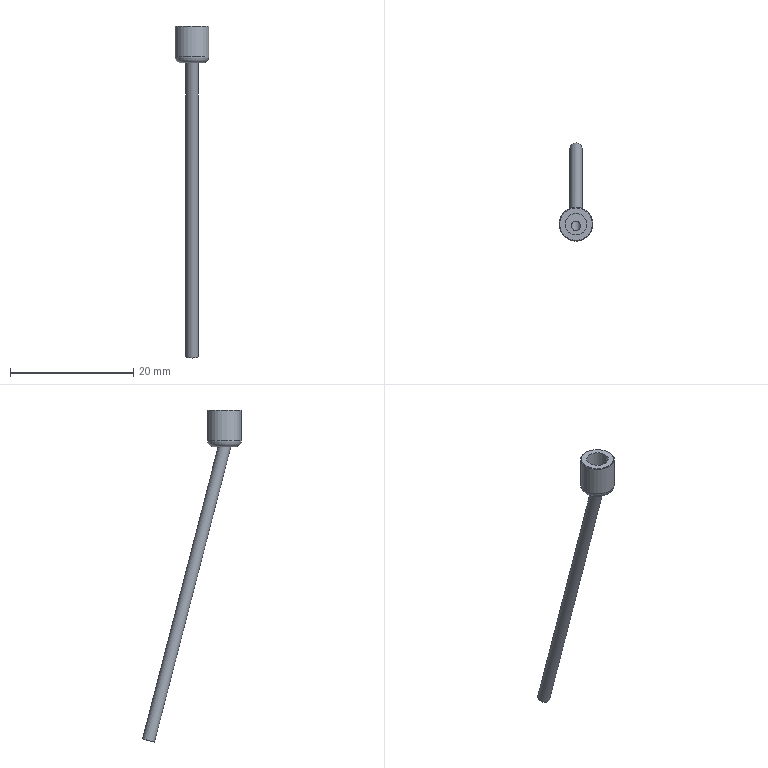Component | NX | AIR_PUMP_PART_01_12 | 1 solid | 10 faces | box 5.5 x 16.05 x 53.95 mm | volume 157 mm3 | plane 4 | cylinder 4 | torus 1 | cone 1 | commonest cylinder face diameters 5.5 x1 2 x1 1.5 x1 3.5 x1
STEP:
#1=CARTESIAN_POINT('',(0.,0.,0.));
#2=DIRECTION('',(0.,0.,1.));
#3=DIRECTION('',(1.,0.,0.));
#4=AXIS2_PLACEMENT_3D('',#1,#2,#3);
#5=CARTESIAN_POINT('',(0.0005589,-29.55,80.052));
#6=VERTEX_POINT('',#5);
#7=CARTESIAN_POINT('',(0.0005589,-32.2,80.052));
#8=DIRECTION('',(0.,0.,1.));
#9=DIRECTION('',(0.,1.,0.));
#10=AXIS2_PLACEMENT_3D('',#7,#8,#9);
#11=CIRCLE('',#10,2.65);
#12=CARTESIAN_POINT('',(0.0005589,-32.2,80.052));
#13=DIRECTION('',(0.,0.,1.));
#14=DIRECTION('',(0.,1.,0.));
#15=AXIS2_PLACEMENT_3D('',#12,#13,#14);
#16=PLANE('',#15);
#17=CARTESIAN_POINT('',(0.,0.));
#18=DIRECTION('',(1.,0.));
#19=AXIS2_PLACEMENT_2D('',#17,#18);
#20=CIRCLE('',#19,2.65);
#21=(GEOMETRIC_REPRESENTATION_CONTEXT(2)PARAMETRIC_REPRESENTATION_CONTEXT()REPRESENTATION_CONTEXT('',''));
#22=DEFINITIONAL_REPRESENTATION('',(#20),#21);
#23=PCURVE('',#16,#22);
#24=CARTESIAN_POINT('',(0.0005589,-32.2,79.952));
#25=DIRECTION('',(0.,0.,-1.));
#26=DIRECTION('',(0.,-1.,0.));
#27=AXIS2_PLACEMENT_3D('',#24,#25,#26);
#28=CONICAL_SURFACE('',#27,2.75,0.7854);
#29=CARTESIAN_POINT('',(9.425,-0.1));
#30=DIRECTION('',(-1.,0.));
#31=VECTOR('',#30,1.);
#32=LINE('',#29,#31);
#33=(GEOMETRIC_REPRESENTATION_CONTEXT(2)PARAMETRIC_REPRESENTATION_CONTEXT()REPRESENTATION_CONTEXT('',''));
#34=DEFINITIONAL_REPRESENTATION('',(#32),#33);
#35=PCURVE('',#28,#34);
#36=SURFACE_CURVE('',#11,(#23,#35),.PCURVE_S1.);
#37=EDGE_CURVE('',#6,#6,#36,.T.);
#38=ORIENTED_EDGE('',*,*,#37,.T.);
#39=EDGE_LOOP('',(#38));
#40=FACE_BOUND('',#39,.T.);
#41=CARTESIAN_POINT('',(0.0005589,-30.45,80.052));
#42=VERTEX_POINT('',#41);
#43=CARTESIAN_POINT('',(0.0005589,-32.2,80.052));
#44=DIRECTION('',(0.,0.,-1.));
#45=DIRECTION('',(-0.,1.,0.));
#46=AXIS2_PLACEMENT_3D('',#43,#44,#45);
#47=CIRCLE('',#46,1.75);
#48=CARTESIAN_POINT('',(1.75,0.));
#49=CARTESIAN_POINT('',(1.75,-3.031));
#50=CARTESIAN_POINT('',(-0.875,-1.516));
#51=CARTESIAN_POINT('',(-3.5,-0.));
#52=CARTESIAN_POINT('',(-0.875,1.516));
#53=CARTESIAN_POINT('',(1.75,3.031));
#54=CARTESIAN_POINT('',(1.75,0.));
#55=(BOUNDED_CURVE()B_SPLINE_CURVE(2,(#48,#49,#50,#51,#52,#53,#54),.UNSPECIFIED.,.T.,.F.)B_SPLINE_CURVE_WITH_KNOTS((1,2,2,2,2,1),(-2.094,0.,2.094,4.189,6.283,8.378),.UNSPECIFIED.)CURVE()GEOMETRIC_REPRESENTATION_ITEM()RATIONAL_B_SPLINE_CURVE((1.,0.5,1.,0.5,1.,0.5,1.))REPRESENTATION_ITEM(''));
#56=(GEOMETRIC_REPRESENTATION_CONTEXT(2)PARAMETRIC_REPRESENTATION_CONTEXT()REPRESENTATION_CONTEXT('',''));
#57=DEFINITIONAL_REPRESENTATION('',(#55),#56);
#58=PCURVE('',#16,#57);
#59=CARTESIAN_POINT('',(0.0005589,-32.2,75.052));
#60=DIRECTION('',(0.,0.,1.));
#61=DIRECTION('',(0.,1.,0.));
#62=AXIS2_PLACEMENT_3D('',#59,#60,#61);
#63=CYLINDRICAL_SURFACE('',#62,1.75);
#64=CARTESIAN_POINT('',(6.283,5.));
#65=DIRECTION('',(-1.,0.));
#66=VECTOR('',#65,1.);
#67=LINE('',#64,#66);
#68=(GEOMETRIC_REPRESENTATION_CONTEXT(2)PARAMETRIC_REPRESENTATION_CONTEXT()REPRESENTATION_CONTEXT('',''));
#69=DEFINITIONAL_REPRESENTATION('',(#67),#68);
#70=PCURVE('',#63,#69);
#71=SURFACE_CURVE('',#47,(#58,#70),.PCURVE_S1.);
#72=EDGE_CURVE('',#42,#42,#71,.T.);
#73=ORIENTED_EDGE('',*,*,#72,.T.);
#74=EDGE_LOOP('',(#73));
#75=FACE_BOUND('',#74,.T.);
#76=ADVANCED_FACE('',(#40,#75),#16,.T.);
#77=CARTESIAN_POINT('',(0.0005589,-33.95,74.052));
#78=VERTEX_POINT('',#77);
#79=CARTESIAN_POINT('',(0.0005589,-32.2,74.052));
#80=DIRECTION('',(0.,0.,-1.));
#81=DIRECTION('',(0.,-1.,0.));
#82=AXIS2_PLACEMENT_3D('',#79,#80,#81);
#83=CIRCLE('',#82,1.75);
#84=CARTESIAN_POINT('',(0.0005589,-32.2,74.052));
#85=DIRECTION('',(0.,0.,-1.));
#86=DIRECTION('',(0.,-1.,0.));
#87=AXIS2_PLACEMENT_3D('',#84,#85,#86);
#88=PLANE('',#87);
#89=CARTESIAN_POINT('',(0.,0.));
#90=DIRECTION('',(1.,0.));
#91=AXIS2_PLACEMENT_2D('',#89,#90);
#92=CIRCLE('',#91,1.75);
#93=(GEOMETRIC_REPRESENTATION_CONTEXT(2)PARAMETRIC_REPRESENTATION_CONTEXT()REPRESENTATION_CONTEXT('',''));
#94=DEFINITIONAL_REPRESENTATION('',(#92),#93);
#95=PCURVE('',#88,#94);
#96=CARTESIAN_POINT('',(0.0005589,-32.2,75.052));
#97=DIRECTION('',(0.,0.,-1.));
#98=DIRECTION('',(0.,-1.,0.));
#99=AXIS2_PLACEMENT_3D('',#96,#97,#98);
#100=TOROIDAL_SURFACE('',#99,1.75,1.);
#101=CARTESIAN_POINT('',(0.,7.854));
#102=DIRECTION('',(1.,0.));
#103=VECTOR('',#102,1.);
#104=LINE('',#101,#103);
#105=(GEOMETRIC_REPRESENTATION_CONTEXT(2)PARAMETRIC_REPRESENTATION_CONTEXT()REPRESENTATION_CONTEXT('',''));
#106=DEFINITIONAL_REPRESENTATION('',(#104),#105);
#107=PCURVE('',#100,#106);
#108=SURFACE_CURVE('',#83,(#95,#107),.PCURVE_S1.);
#109=EDGE_CURVE('',#78,#78,#108,.T.);
#110=ORIENTED_EDGE('',*,*,#109,.T.);
#111=EDGE_LOOP('',(#110));
#112=FACE_BOUND('',#111,.T.);
#113=CARTESIAN_POINT('',(0.0005589,-31.167,74.052));
#114=VERTEX_POINT('',#113);
#115=CARTESIAN_POINT('',(0.0005589,-33.233,74.052));
#116=VERTEX_POINT('',#115);
#117=CARTESIAN_POINT('',(0.0005589,-32.2,74.052));
#118=DIRECTION('',(0.,0.,-1.));
#119=DIRECTION('',(0.,1.,0.));
#120=AXIS2_PLACEMENT_3D('',#117,#118,#119);
#121=ELLIPSE('',#120,1.033,1.);
#122=CARTESIAN_POINT('',(0.,0.));
#123=DIRECTION('',(-1.,0.));
#124=AXIS2_PLACEMENT_2D('',#122,#123);
#125=ELLIPSE('',#124,1.033,1.);
#126=(GEOMETRIC_REPRESENTATION_CONTEXT(2)PARAMETRIC_REPRESENTATION_CONTEXT()REPRESENTATION_CONTEXT('',''));
#127=DEFINITIONAL_REPRESENTATION('',(#125),#126);
#128=PCURVE('',#88,#127);
#129=CARTESIAN_POINT('',(0.0005589,-32.2,74.052));
#130=DIRECTION('',(0.,0.2504,-0.9681));
#131=DIRECTION('',(0.,-0.9681,-0.2504));
#132=AXIS2_PLACEMENT_3D('',#129,#130,#131);
#133=CYLINDRICAL_SURFACE('',#132,1.);
#134=CARTESIAN_POINT('',(3.142,0.2586));
#135=CARTESIAN_POINT('',(3.237,0.2588));
#136=CARTESIAN_POINT('',(3.427,0.2515));
#137=CARTESIAN_POINT('',(3.713,0.2206));
#138=CARTESIAN_POINT('',(3.998,0.1717));
#139=CARTESIAN_POINT('',(4.284,0.1089));
#140=CARTESIAN_POINT('',(4.57,0.03731));
#141=CARTESIAN_POINT('',(4.855,-0.03731));
#142=CARTESIAN_POINT('',(5.141,-0.1089));
#143=CARTESIAN_POINT('',(5.426,-0.1717));
#144=CARTESIAN_POINT('',(5.712,-0.2205));
#145=CARTESIAN_POINT('',(5.998,-0.2515));
#146=CARTESIAN_POINT('',(6.283,-0.2622));
#147=CARTESIAN_POINT('',(6.569,-0.2515));
#148=CARTESIAN_POINT('',(6.854,-0.2205));
#149=CARTESIAN_POINT('',(7.14,-0.1717));
#150=CARTESIAN_POINT('',(7.426,-0.1089));
#151=CARTESIAN_POINT('',(7.711,-0.03731));
#152=CARTESIAN_POINT('',(7.997,0.03731));
#153=CARTESIAN_POINT('',(8.282,0.1089));
#154=CARTESIAN_POINT('',(8.568,0.1717));
#155=CARTESIAN_POINT('',(8.854,0.2206));
#156=CARTESIAN_POINT('',(9.139,0.2515));
#157=CARTESIAN_POINT('',(9.33,0.2588));
#158=CARTESIAN_POINT('',(9.425,0.2586));
#159=B_SPLINE_CURVE_WITH_KNOTS('',3,(#134,#135,#136,#137,#138,#139,#140,#141,#142,#143,#144,#145,#146,#147,#148,#149,#150,#151,#152,#153,#154,#155,#156,#157,#158),.UNSPECIFIED.,.F.,.F.,(4,1,1,1,1,1,1,1,1,1,1,1,1,1,1,1,1,1,1,1,1,1,4),(0.,0.2856,0.5712,0.8568,1.142,1.428,1.714,1.999,2.285,2.57,2.856,3.142,3.427,3.713,3.998,4.284,4.57,4.855,5.141,5.426,5.712,5.998,6.283),.QUASI_UNIFORM_KNOTS.);
#160=(GEOMETRIC_REPRESENTATION_CONTEXT(2)PARAMETRIC_REPRESENTATION_CONTEXT()REPRESENTATION_CONTEXT('',''));
#161=DEFINITIONAL_REPRESENTATION('',(#159),#160);
#162=PCURVE('',#133,#161);
#163=SURFACE_CURVE('',#121,(#128,#162),.PCURVE_S1.);
#164=EDGE_CURVE('',#114,#116,#163,.T.);
#165=ORIENTED_EDGE('',*,*,#164,.F.);
#166=CARTESIAN_POINT('',(0.0005589,-32.2,74.052));
#167=DIRECTION('',(0.,0.,-1.));
#168=DIRECTION('',(0.,1.,0.));
#169=AXIS2_PLACEMENT_3D('',#166,#167,#168);
#170=ELLIPSE('',#169,1.033,1.);
#171=CARTESIAN_POINT('',(0.,0.));
#172=DIRECTION('',(-1.,0.));
#173=AXIS2_PLACEMENT_2D('',#171,#172);
#174=ELLIPSE('',#173,1.033,1.);
#175=(GEOMETRIC_REPRESENTATION_CONTEXT(2)PARAMETRIC_REPRESENTATION_CONTEXT()REPRESENTATION_CONTEXT('',''));
#176=DEFINITIONAL_REPRESENTATION('',(#174),#175);
#177=PCURVE('',#88,#176);
#178=CARTESIAN_POINT('',(-3.142,0.2586));
#179=CARTESIAN_POINT('',(-3.046,0.2588));
#180=CARTESIAN_POINT('',(-2.856,0.2515));
#181=CARTESIAN_POINT('',(-2.57,0.2206));
#182=CARTESIAN_POINT('',(-2.285,0.1717));
#183=CARTESIAN_POINT('',(-1.999,0.1089));
#184=CARTESIAN_POINT('',(-1.714,0.03731));
#185=CARTESIAN_POINT('',(-1.428,-0.03731));
#186=CARTESIAN_POINT('',(-1.142,-0.1089));
#187=CARTESIAN_POINT('',(-0.8568,-0.1717));
#188=CARTESIAN_POINT('',(-0.5712,-0.2205));
#189=CARTESIAN_POINT('',(-0.2856,-0.2515));
#190=CARTESIAN_POINT('',(0.,-0.2622));
#191=CARTESIAN_POINT('',(0.2856,-0.2515));
#192=CARTESIAN_POINT('',(0.5712,-0.2205));
#193=CARTESIAN_POINT('',(0.8568,-0.1717));
#194=CARTESIAN_POINT('',(1.142,-0.1089));
#195=CARTESIAN_POINT('',(1.428,-0.03731));
#196=CARTESIAN_POINT('',(1.714,0.03731));
#197=CARTESIAN_POINT('',(1.999,0.1089));
#198=CARTESIAN_POINT('',(2.285,0.1717));
#199=CARTESIAN_POINT('',(2.57,0.2206));
#200=CARTESIAN_POINT('',(2.856,0.2515));
#201=CARTESIAN_POINT('',(3.046,0.2588));
#202=CARTESIAN_POINT('',(3.142,0.2586));
#203=B_SPLINE_CURVE_WITH_KNOTS('',3,(#178,#179,#180,#181,#182,#183,#184,#185,#186,#187,#188,#189,#190,#191,#192,#193,#194,#195,#196,#197,#198,#199,#200,#201,#202),.UNSPECIFIED.,.F.,.F.,(4,1,1,1,1,1,1,1,1,1,1,1,1,1,1,1,1,1,1,1,1,1,4),(0.,0.2856,0.5712,0.8568,1.142,1.428,1.714,1.999,2.285,2.57,2.856,3.142,3.427,3.713,3.998,4.284,4.57,4.855,5.141,5.426,5.712,5.998,6.283),.QUASI_UNIFORM_KNOTS.);
#204=(GEOMETRIC_REPRESENTATION_CONTEXT(2)PARAMETRIC_REPRESENTATION_CONTEXT()REPRESENTATION_CONTEXT('',''));
#205=DEFINITIONAL_REPRESENTATION('',(#203),#204);
#206=PCURVE('',#133,#205);
#207=SURFACE_CURVE('',#170,(#177,#206),.PCURVE_S1.);
#208=EDGE_CURVE('',#116,#114,#207,.T.);
#209=ORIENTED_EDGE('',*,*,#208,.F.);
#210=EDGE_LOOP('',(#165,#209));
#211=FACE_BOUND('',#210,.T.);
#212=ADVANCED_FACE('',(#112,#211),#88,.T.);
#213=CARTESIAN_POINT('',(0.0005589,-29.45,79.952));
#214=VERTEX_POINT('',#213);
#215=CARTESIAN_POINT('',(0.0005589,-32.2,79.952));
#216=DIRECTION('',(0.,0.,-1.));
#217=DIRECTION('',(0.,1.,0.));
#218=AXIS2_PLACEMENT_3D('',#215,#216,#217);
#219=CIRCLE('',#218,2.75);
#220=CARTESIAN_POINT('',(0.0005589,-32.2,74.052));
#221=DIRECTION('',(0.,0.,1.));
#222=DIRECTION('',(0.,1.,0.));
#223=AXIS2_PLACEMENT_3D('',#220,#221,#222);
#224=CYLINDRICAL_SURFACE('',#223,2.75);
#225=CARTESIAN_POINT('',(6.283,5.9));
#226=DIRECTION('',(-1.,0.));
#227=VECTOR('',#226,1.);
#228=LINE('',#225,#227);
#229=(GEOMETRIC_REPRESENTATION_CONTEXT(2)PARAMETRIC_REPRESENTATION_CONTEXT()REPRESENTATION_CONTEXT('',''));
#230=DEFINITIONAL_REPRESENTATION('',(#228),#229);
#231=PCURVE('',#224,#230);
#232=CARTESIAN_POINT('',(3.142,0.));
#233=DIRECTION('',(1.,0.));
#234=VECTOR('',#233,1.);
#235=LINE('',#232,#234);
#236=(GEOMETRIC_REPRESENTATION_CONTEXT(2)PARAMETRIC_REPRESENTATION_CONTEXT()REPRESENTATION_CONTEXT('',''));
#237=DEFINITIONAL_REPRESENTATION('',(#235),#236);
#238=PCURVE('',#28,#237);
#239=SURFACE_CURVE('',#219,(#231,#238),.PCURVE_S1.);
#240=EDGE_CURVE('',#214,#214,#239,.T.);
#241=ORIENTED_EDGE('',*,*,#240,.T.);
#242=CARTESIAN_POINT('',(0.0005589,-29.45,75.052));
#243=VERTEX_POINT('',#242);
#244=CARTESIAN_POINT('',(0.0005589,-29.45,75.052));
#245=CARTESIAN_POINT('',(0.0005589,-29.45,79.952));
#246=B_SPLINE_CURVE_WITH_KNOTS('',1,(#244,#245),.UNSPECIFIED.,.F.,.F.,(2,2),(1.,5.9),.PIECEWISE_BEZIER_KNOTS.);
#247=CARTESIAN_POINT('',(0.,0.));
#248=DIRECTION('',(0.,1.));
#249=VECTOR('',#248,1.);
#250=LINE('',#247,#249);
#251=(GEOMETRIC_REPRESENTATION_CONTEXT(2)PARAMETRIC_REPRESENTATION_CONTEXT()REPRESENTATION_CONTEXT('',''));
#252=DEFINITIONAL_REPRESENTATION('',(#250),#251);
#253=PCURVE('',#224,#252);
#254=CARTESIAN_POINT('',(6.283,0.));
#255=DIRECTION('',(0.,1.));
#256=VECTOR('',#255,1.);
#257=LINE('',#254,#256);
#258=(GEOMETRIC_REPRESENTATION_CONTEXT(2)PARAMETRIC_REPRESENTATION_CONTEXT()REPRESENTATION_CONTEXT('',''));
#259=DEFINITIONAL_REPRESENTATION('',(#257),#258);
#260=PCURVE('',#224,#259);
#261=SEAM_CURVE('',#246,(#253,#260),.PCURVE_S1.);
#262=EDGE_CURVE('',#243,#214,#261,.T.);
#263=ORIENTED_EDGE('',*,*,#262,.F.);
#264=CARTESIAN_POINT('',(0.0005589,-34.95,75.052));
#265=VERTEX_POINT('',#264);
#266=CARTESIAN_POINT('',(0.0005589,-32.2,75.052));
#267=DIRECTION('',(0.,0.,1.));
#268=DIRECTION('',(0.,-1.,0.));
#269=AXIS2_PLACEMENT_3D('',#266,#267,#268);
#270=CIRCLE('',#269,2.75);
#271=CARTESIAN_POINT('',(-3.142,1.));
#272=DIRECTION('',(1.,0.));
#273=VECTOR('',#272,1.);
#274=LINE('',#271,#273);
#275=(GEOMETRIC_REPRESENTATION_CONTEXT(2)PARAMETRIC_REPRESENTATION_CONTEXT()REPRESENTATION_CONTEXT('',''));
#276=DEFINITIONAL_REPRESENTATION('',(#274),#275);
#277=PCURVE('',#224,#276);
#278=CARTESIAN_POINT('',(6.283,6.283));
#279=DIRECTION('',(-1.,0.));
#280=VECTOR('',#279,1.);
#281=LINE('',#278,#280);
#282=(GEOMETRIC_REPRESENTATION_CONTEXT(2)PARAMETRIC_REPRESENTATION_CONTEXT()REPRESENTATION_CONTEXT('',''));
#283=DEFINITIONAL_REPRESENTATION('',(#281),#282);
#284=PCURVE('',#100,#283);
#285=SURFACE_CURVE('',#270,(#277,#284),.PCURVE_S1.);
#286=EDGE_CURVE('',#243,#265,#285,.T.);
#287=ORIENTED_EDGE('',*,*,#286,.T.);
#288=CARTESIAN_POINT('',(0.0005589,-32.2,75.052));
#289=DIRECTION('',(0.,0.,1.));
#290=DIRECTION('',(0.,-1.,0.));
#291=AXIS2_PLACEMENT_3D('',#288,#289,#290);
#292=CIRCLE('',#291,2.75);
#293=CARTESIAN_POINT('',(3.142,1.));
#294=DIRECTION('',(1.,0.));
#295=VECTOR('',#294,1.);
#296=LINE('',#293,#295);
#297=(GEOMETRIC_REPRESENTATION_CONTEXT(2)PARAMETRIC_REPRESENTATION_CONTEXT()REPRESENTATION_CONTEXT('',''));
#298=DEFINITIONAL_REPRESENTATION('',(#296),#297);
#299=PCURVE('',#224,#298);
#300=CARTESIAN_POINT('',(6.283,6.283));
#301=DIRECTION('',(-1.,0.));
#302=VECTOR('',#301,1.);
#303=LINE('',#300,#302);
#304=(GEOMETRIC_REPRESENTATION_CONTEXT(2)PARAMETRIC_REPRESENTATION_CONTEXT()REPRESENTATION_CONTEXT('',''));
#305=DEFINITIONAL_REPRESENTATION('',(#303),#304);
#306=PCURVE('',#100,#305);
#307=SURFACE_CURVE('',#292,(#299,#306),.PCURVE_S1.);
#308=EDGE_CURVE('',#265,#243,#307,.T.);
#309=ORIENTED_EDGE('',*,*,#308,.T.);
#310=ORIENTED_EDGE('',*,*,#262,.T.);
#311=EDGE_LOOP('',(#241,#263,#287,#309,#310));
#312=FACE_BOUND('',#311,.T.);
#313=ADVANCED_FACE('',(#312),#224,.T.);
#314=ORIENTED_EDGE('',*,*,#164,.T.);
#315=CARTESIAN_POINT('',(0.0005589,-20.832,26.101));
#316=VERTEX_POINT('',#315);
#317=CARTESIAN_POINT('',(0.0005589,-33.233,74.052));
#318=CARTESIAN_POINT('',(0.0005589,-20.832,26.101));
#319=B_SPLINE_CURVE_WITH_KNOTS('',1,(#317,#318),.UNSPECIFIED.,.F.,.F.,(2,2),(-0.2586,49.269),.PIECEWISE_BEZIER_KNOTS.);
#320=CARTESIAN_POINT('',(6.283,0.));
#321=DIRECTION('',(0.,1.));
#322=VECTOR('',#321,1.);
#323=LINE('',#320,#322);
#324=(GEOMETRIC_REPRESENTATION_CONTEXT(2)PARAMETRIC_REPRESENTATION_CONTEXT()REPRESENTATION_CONTEXT('',''));
#325=DEFINITIONAL_REPRESENTATION('',(#323),#324);
#326=PCURVE('',#133,#325);
#327=CARTESIAN_POINT('',(0.,0.));
#328=DIRECTION('',(0.,1.));
#329=VECTOR('',#328,1.);
#330=LINE('',#327,#329);
#331=(GEOMETRIC_REPRESENTATION_CONTEXT(2)PARAMETRIC_REPRESENTATION_CONTEXT()REPRESENTATION_CONTEXT('',''));
#332=DEFINITIONAL_REPRESENTATION('',(#330),#331);
#333=PCURVE('',#133,#332);
#334=SEAM_CURVE('',#319,(#326,#333),.PCURVE_S1.);
#335=EDGE_CURVE('',#116,#316,#334,.T.);
#336=ORIENTED_EDGE('',*,*,#335,.T.);
#337=CARTESIAN_POINT('',(0.0005589,-19.864,26.352));
#338=DIRECTION('',(0.,0.2504,-0.9681));
#339=DIRECTION('',(0.,-0.9681,-0.2504));
#340=AXIS2_PLACEMENT_3D('',#337,#338,#339);
#341=CIRCLE('',#340,1.);
#342=CARTESIAN_POINT('',(0.,49.269));
#343=DIRECTION('',(1.,0.));
#344=VECTOR('',#343,1.);
#345=LINE('',#342,#344);
#346=(GEOMETRIC_REPRESENTATION_CONTEXT(2)PARAMETRIC_REPRESENTATION_CONTEXT()REPRESENTATION_CONTEXT('',''));
#347=DEFINITIONAL_REPRESENTATION('',(#345),#346);
#348=PCURVE('',#133,#347);
#349=CARTESIAN_POINT('',(0.0005589,-19.864,26.352));
#350=DIRECTION('',(0.,0.2504,-0.9681));
#351=DIRECTION('',(0.,-0.9681,-0.2504));
#352=AXIS2_PLACEMENT_3D('',#349,#350,#351);
#353=PLANE('',#352);
#354=CARTESIAN_POINT('',(0.,0.));
#355=DIRECTION('',(1.,0.));
#356=AXIS2_PLACEMENT_2D('',#354,#355);
#357=CIRCLE('',#356,1.);
#358=(GEOMETRIC_REPRESENTATION_CONTEXT(2)PARAMETRIC_REPRESENTATION_CONTEXT()REPRESENTATION_CONTEXT('',''));
#359=DEFINITIONAL_REPRESENTATION('',(#357),#358);
#360=PCURVE('',#353,#359);
#361=SURFACE_CURVE('',#341,(#348,#360),.PCURVE_S1.);
#362=EDGE_CURVE('',#316,#316,#361,.T.);
#363=ORIENTED_EDGE('',*,*,#362,.F.);
#364=ORIENTED_EDGE('',*,*,#335,.F.);
#365=ORIENTED_EDGE('',*,*,#208,.T.);
#366=EDGE_LOOP('',(#314,#336,#363,#364,#365));
#367=FACE_BOUND('',#366,.T.);
#368=ADVANCED_FACE('',(#367),#133,.T.);
#369=CARTESIAN_POINT('',(0.0005589,-20.59,26.164));
#370=VERTEX_POINT('',#369);
#371=CARTESIAN_POINT('',(0.0005589,-19.864,26.352));
#372=DIRECTION('',(0.,0.2504,-0.9681));
#373=DIRECTION('',(0.,-0.9681,-0.2504));
#374=AXIS2_PLACEMENT_3D('',#371,#372,#373);
#375=CIRCLE('',#374,0.75);
#376=CARTESIAN_POINT('',(-0.,0.));
#377=DIRECTION('',(1.,0.));
#378=AXIS2_PLACEMENT_2D('',#376,#377);
#379=CIRCLE('',#378,0.75);
#380=(GEOMETRIC_REPRESENTATION_CONTEXT(2)PARAMETRIC_REPRESENTATION_CONTEXT()REPRESENTATION_CONTEXT('',''));
#381=DEFINITIONAL_REPRESENTATION('',(#379),#380);
#382=PCURVE('',#353,#381);
#383=CARTESIAN_POINT('',(0.0005589,-32.733,76.115));
#384=DIRECTION('',(0.,0.2504,-0.9681));
#385=DIRECTION('',(0.,-0.9681,-0.2504));
#386=AXIS2_PLACEMENT_3D('',#383,#384,#385);
#387=CYLINDRICAL_SURFACE('',#386,0.75);
#388=CARTESIAN_POINT('',(0.,51.4));
#389=DIRECTION('',(1.,0.));
#390=VECTOR('',#389,1.);
#391=LINE('',#388,#390);
#392=(GEOMETRIC_REPRESENTATION_CONTEXT(2)PARAMETRIC_REPRESENTATION_CONTEXT()REPRESENTATION_CONTEXT('',''));
#393=DEFINITIONAL_REPRESENTATION('',(#391),#392);
#394=PCURVE('',#387,#393);
#395=SURFACE_CURVE('',#375,(#382,#394),.PCURVE_S1.);
#396=EDGE_CURVE('',#370,#370,#395,.T.);
#397=ORIENTED_EDGE('',*,*,#396,.F.);
#398=EDGE_LOOP('',(#397));
#399=FACE_BOUND('',#398,.T.);
#400=ORIENTED_EDGE('',*,*,#362,.T.);
#401=EDGE_LOOP('',(#400));
#402=FACE_BOUND('',#401,.T.);
#403=ADVANCED_FACE('',(#399,#402),#353,.T.);
#404=CARTESIAN_POINT('',(0.0005589,-33.233,75.052));
#405=VERTEX_POINT('',#404);
#406=CARTESIAN_POINT('',(0.0005589,-31.684,75.052));
#407=VERTEX_POINT('',#406);
#408=CARTESIAN_POINT('',(0.0005589,-32.459,75.052));
#409=DIRECTION('',(0.,0.,1.));
#410=DIRECTION('',(0.,1.,0.));
#411=AXIS2_PLACEMENT_3D('',#408,#409,#410);
#412=ELLIPSE('',#411,0.7747,0.75);
#413=CARTESIAN_POINT('',(9.425,1.292));
#414=CARTESIAN_POINT('',(9.33,1.292));
#415=CARTESIAN_POINT('',(9.139,1.286));
#416=CARTESIAN_POINT('',(8.854,1.263));
#417=CARTESIAN_POINT('',(8.568,1.227));
#418=CARTESIAN_POINT('',(8.282,1.179));
#419=CARTESIAN_POINT('',(7.997,1.126));
#420=CARTESIAN_POINT('',(7.711,1.07));
#421=CARTESIAN_POINT('',(7.426,1.016));
#422=CARTESIAN_POINT('',(7.14,0.969));
#423=CARTESIAN_POINT('',(6.854,0.9323));
#424=CARTESIAN_POINT('',(6.569,0.9091));
#425=CARTESIAN_POINT('',(6.283,0.9011));
#426=CARTESIAN_POINT('',(5.998,0.9091));
#427=CARTESIAN_POINT('',(5.712,0.9323));
#428=CARTESIAN_POINT('',(5.426,0.969));
#429=CARTESIAN_POINT('',(5.141,1.016));
#430=CARTESIAN_POINT('',(4.855,1.07));
#431=CARTESIAN_POINT('',(4.57,1.126));
#432=CARTESIAN_POINT('',(4.284,1.179));
#433=CARTESIAN_POINT('',(3.998,1.227));
#434=CARTESIAN_POINT('',(3.713,1.263));
#435=CARTESIAN_POINT('',(3.427,1.286));
#436=CARTESIAN_POINT('',(3.237,1.292));
#437=CARTESIAN_POINT('',(3.142,1.292));
#438=B_SPLINE_CURVE_WITH_KNOTS('',3,(#413,#414,#415,#416,#417,#418,#419,#420,#421,#422,#423,#424,#425,#426,#427,#428,#429,#430,#431,#432,#433,#434,#435,#436,#437),.UNSPECIFIED.,.F.,.F.,(4,1,1,1,1,1,1,1,1,1,1,1,1,1,1,1,1,1,1,1,1,1,4),(0.,0.2856,0.5712,0.8568,1.142,1.428,1.714,1.999,2.285,2.57,2.856,3.142,3.427,3.713,3.998,4.284,4.57,4.855,5.141,5.426,5.712,5.998,6.283),.QUASI_UNIFORM_KNOTS.);
#439=(GEOMETRIC_REPRESENTATION_CONTEXT(2)PARAMETRIC_REPRESENTATION_CONTEXT()REPRESENTATION_CONTEXT('',''));
#440=DEFINITIONAL_REPRESENTATION('',(#438),#439);
#441=PCURVE('',#387,#440);
#442=CARTESIAN_POINT('',(0.0005589,-32.2,75.052));
#443=DIRECTION('',(0.,0.,-1.));
#444=DIRECTION('',(0.,-1.,0.));
#445=AXIS2_PLACEMENT_3D('',#442,#443,#444);
#446=PLANE('',#445);
#447=CARTESIAN_POINT('',(-0.5161,0.));
#448=CARTESIAN_POINT('',(-0.5161,1.299));
#449=CARTESIAN_POINT('',(0.646,0.6495));
#450=CARTESIAN_POINT('',(1.808,0.));
#451=CARTESIAN_POINT('',(0.646,-0.6495));
#452=CARTESIAN_POINT('',(-0.5161,-1.299));
#453=CARTESIAN_POINT('',(-0.5161,0.));
#454=(BOUNDED_CURVE()B_SPLINE_CURVE(2,(#447,#448,#449,#450,#451,#452,#453),.UNSPECIFIED.,.T.,.F.)B_SPLINE_CURVE_WITH_KNOTS((1,2,2,2,2,1),(-2.094,0.,2.094,4.189,6.283,8.378),.UNSPECIFIED.)CURVE()GEOMETRIC_REPRESENTATION_ITEM()RATIONAL_B_SPLINE_CURVE((1.,0.5,1.,0.5,1.,0.5,1.))REPRESENTATION_ITEM(''));
#455=(GEOMETRIC_REPRESENTATION_CONTEXT(2)PARAMETRIC_REPRESENTATION_CONTEXT()REPRESENTATION_CONTEXT('',''));
#456=DEFINITIONAL_REPRESENTATION('',(#454),#455);
#457=PCURVE('',#446,#456);
#458=SURFACE_CURVE('',#412,(#441,#457),.PCURVE_S1.);
#459=EDGE_CURVE('',#405,#407,#458,.T.);
#460=ORIENTED_EDGE('',*,*,#459,.F.);
#461=CARTESIAN_POINT('',(0.0005589,-33.233,75.052));
#462=CARTESIAN_POINT('',(0.0005589,-20.59,26.164));
#463=B_SPLINE_CURVE_WITH_KNOTS('',1,(#461,#462),.UNSPECIFIED.,.F.,.F.,(2,2),(0.9038,51.4),.PIECEWISE_BEZIER_KNOTS.);
#464=CARTESIAN_POINT('',(6.283,0.));
#465=DIRECTION('',(0.,1.));
#466=VECTOR('',#465,1.);
#467=LINE('',#464,#466);
#468=(GEOMETRIC_REPRESENTATION_CONTEXT(2)PARAMETRIC_REPRESENTATION_CONTEXT()REPRESENTATION_CONTEXT('',''));
#469=DEFINITIONAL_REPRESENTATION('',(#467),#468);
#470=PCURVE('',#387,#469);
#471=CARTESIAN_POINT('',(0.,0.));
#472=DIRECTION('',(0.,1.));
#473=VECTOR('',#472,1.);
#474=LINE('',#471,#473);
#475=(GEOMETRIC_REPRESENTATION_CONTEXT(2)PARAMETRIC_REPRESENTATION_CONTEXT()REPRESENTATION_CONTEXT('',''));
#476=DEFINITIONAL_REPRESENTATION('',(#474),#475);
#477=PCURVE('',#387,#476);
#478=SEAM_CURVE('',#463,(#470,#477),.PCURVE_S1.);
#479=EDGE_CURVE('',#405,#370,#478,.T.);
#480=ORIENTED_EDGE('',*,*,#479,.T.);
#481=ORIENTED_EDGE('',*,*,#396,.F.);
#482=ORIENTED_EDGE('',*,*,#479,.F.);
#483=CARTESIAN_POINT('',(0.0005589,-32.459,75.052));
#484=DIRECTION('',(0.,0.,1.));
#485=DIRECTION('',(0.,1.,0.));
#486=AXIS2_PLACEMENT_3D('',#483,#484,#485);
#487=ELLIPSE('',#486,0.7747,0.75);
#488=CARTESIAN_POINT('',(3.142,1.292));
#489=CARTESIAN_POINT('',(3.046,1.292));
#490=CARTESIAN_POINT('',(2.856,1.286));
#491=CARTESIAN_POINT('',(2.57,1.263));
#492=CARTESIAN_POINT('',(2.285,1.227));
#493=CARTESIAN_POINT('',(1.999,1.179));
#494=CARTESIAN_POINT('',(1.714,1.126));
#495=CARTESIAN_POINT('',(1.428,1.07));
#496=CARTESIAN_POINT('',(1.142,1.016));
#497=CARTESIAN_POINT('',(0.8568,0.969));
#498=CARTESIAN_POINT('',(0.5712,0.9323));
#499=CARTESIAN_POINT('',(0.2856,0.9091));
#500=CARTESIAN_POINT('',(0.,0.9011));
#501=CARTESIAN_POINT('',(-0.2856,0.9091));
#502=CARTESIAN_POINT('',(-0.5712,0.9323));
#503=CARTESIAN_POINT('',(-0.8568,0.969));
#504=CARTESIAN_POINT('',(-1.142,1.016));
#505=CARTESIAN_POINT('',(-1.428,1.07));
#506=CARTESIAN_POINT('',(-1.714,1.126));
#507=CARTESIAN_POINT('',(-1.999,1.179));
#508=CARTESIAN_POINT('',(-2.285,1.227));
#509=CARTESIAN_POINT('',(-2.57,1.263));
#510=CARTESIAN_POINT('',(-2.856,1.286));
#511=CARTESIAN_POINT('',(-3.046,1.292));
#512=CARTESIAN_POINT('',(-3.142,1.292));
#513=B_SPLINE_CURVE_WITH_KNOTS('',3,(#488,#489,#490,#491,#492,#493,#494,#495,#496,#497,#498,#499,#500,#501,#502,#503,#504,#505,#506,#507,#508,#509,#510,#511,#512),.UNSPECIFIED.,.F.,.F.,(4,1,1,1,1,1,1,1,1,1,1,1,1,1,1,1,1,1,1,1,1,1,4),(0.,0.2856,0.5712,0.8568,1.142,1.428,1.714,1.999,2.285,2.57,2.856,3.142,3.427,3.713,3.998,4.284,4.57,4.855,5.141,5.426,5.712,5.998,6.283),.QUASI_UNIFORM_KNOTS.);
#514=(GEOMETRIC_REPRESENTATION_CONTEXT(2)PARAMETRIC_REPRESENTATION_CONTEXT()REPRESENTATION_CONTEXT('',''));
#515=DEFINITIONAL_REPRESENTATION('',(#513),#514);
#516=PCURVE('',#387,#515);
#517=CARTESIAN_POINT('',(-0.5161,0.));
#518=CARTESIAN_POINT('',(-0.5161,1.299));
#519=CARTESIAN_POINT('',(0.646,0.6495));
#520=CARTESIAN_POINT('',(1.808,0.));
#521=CARTESIAN_POINT('',(0.646,-0.6495));
#522=CARTESIAN_POINT('',(-0.5161,-1.299));
#523=CARTESIAN_POINT('',(-0.5161,0.));
#524=(BOUNDED_CURVE()B_SPLINE_CURVE(2,(#517,#518,#519,#520,#521,#522,#523),.UNSPECIFIED.,.T.,.F.)B_SPLINE_CURVE_WITH_KNOTS((1,2,2,2,2,1),(-2.094,0.,2.094,4.189,6.283,8.378),.UNSPECIFIED.)CURVE()GEOMETRIC_REPRESENTATION_ITEM()RATIONAL_B_SPLINE_CURVE((1.,0.5,1.,0.5,1.,0.5,1.))REPRESENTATION_ITEM(''));
#525=(GEOMETRIC_REPRESENTATION_CONTEXT(2)PARAMETRIC_REPRESENTATION_CONTEXT()REPRESENTATION_CONTEXT('',''));
#526=DEFINITIONAL_REPRESENTATION('',(#524),#525);
#527=PCURVE('',#446,#526);
#528=SURFACE_CURVE('',#487,(#516,#527),.PCURVE_S1.);
#529=EDGE_CURVE('',#407,#405,#528,.T.);
#530=ORIENTED_EDGE('',*,*,#529,.F.);
#531=EDGE_LOOP('',(#460,#480,#481,#482,#530));
#532=FACE_BOUND('',#531,.F.);
#533=ADVANCED_FACE('',(#532),#387,.F.);
#534=CARTESIAN_POINT('',(0.0005589,-30.45,75.052));
#535=VERTEX_POINT('',#534);
#536=CARTESIAN_POINT('',(0.0005589,-32.2,75.052));
#537=DIRECTION('',(0.,0.,1.));
#538=DIRECTION('',(-0.,1.,0.));
#539=AXIS2_PLACEMENT_3D('',#536,#537,#538);
#540=CIRCLE('',#539,1.75);
#541=CARTESIAN_POINT('',(-1.75,0.));
#542=CARTESIAN_POINT('',(-1.75,3.031));
#543=CARTESIAN_POINT('',(0.875,1.516));
#544=CARTESIAN_POINT('',(3.5,0.));
#545=CARTESIAN_POINT('',(0.875,-1.516));
#546=CARTESIAN_POINT('',(-1.75,-3.031));
#547=CARTESIAN_POINT('',(-1.75,0.));
#548=(BOUNDED_CURVE()B_SPLINE_CURVE(2,(#541,#542,#543,#544,#545,#546,#547),.UNSPECIFIED.,.T.,.F.)B_SPLINE_CURVE_WITH_KNOTS((1,2,2,2,2,1),(-2.094,0.,2.094,4.189,6.283,8.378),.UNSPECIFIED.)CURVE()GEOMETRIC_REPRESENTATION_ITEM()RATIONAL_B_SPLINE_CURVE((1.,0.5,1.,0.5,1.,0.5,1.))REPRESENTATION_ITEM(''));
#549=(GEOMETRIC_REPRESENTATION_CONTEXT(2)PARAMETRIC_REPRESENTATION_CONTEXT()REPRESENTATION_CONTEXT('',''));
#550=DEFINITIONAL_REPRESENTATION('',(#548),#549);
#551=PCURVE('',#446,#550);
#552=CARTESIAN_POINT('',(0.,0.));
#553=DIRECTION('',(1.,0.));
#554=VECTOR('',#553,1.);
#555=LINE('',#552,#554);
#556=(GEOMETRIC_REPRESENTATION_CONTEXT(2)PARAMETRIC_REPRESENTATION_CONTEXT()REPRESENTATION_CONTEXT('',''));
#557=DEFINITIONAL_REPRESENTATION('',(#555),#556);
#558=PCURVE('',#63,#557);
#559=SURFACE_CURVE('',#540,(#551,#558),.PCURVE_S1.);
#560=EDGE_CURVE('',#535,#535,#559,.T.);
#561=ORIENTED_EDGE('',*,*,#560,.T.);
#562=EDGE_LOOP('',(#561));
#563=FACE_BOUND('',#562,.T.);
#564=ORIENTED_EDGE('',*,*,#529,.F.);
#565=ORIENTED_EDGE('',*,*,#459,.F.);
#566=EDGE_LOOP('',(#564,#565));
#567=FACE_BOUND('',#566,.T.);
#568=ADVANCED_FACE('',(#563,#567),#446,.F.);
#569=ORIENTED_EDGE('',*,*,#560,.T.);
#570=CARTESIAN_POINT('',(0.0005589,-30.45,75.052));
#571=CARTESIAN_POINT('',(0.0005589,-30.45,80.052));
#572=B_SPLINE_CURVE_WITH_KNOTS('',1,(#570,#571),.UNSPECIFIED.,.F.,.F.,(2,2),(0.,5.),.PIECEWISE_BEZIER_KNOTS.);
#573=CARTESIAN_POINT('',(6.283,0.));
#574=DIRECTION('',(0.,1.));
#575=VECTOR('',#574,1.);
#576=LINE('',#573,#575);
#577=(GEOMETRIC_REPRESENTATION_CONTEXT(2)PARAMETRIC_REPRESENTATION_CONTEXT()REPRESENTATION_CONTEXT('',''));
#578=DEFINITIONAL_REPRESENTATION('',(#576),#577);
#579=PCURVE('',#63,#578);
#580=CARTESIAN_POINT('',(0.,0.));
#581=DIRECTION('',(0.,1.));
#582=VECTOR('',#581,1.);
#583=LINE('',#580,#582);
#584=(GEOMETRIC_REPRESENTATION_CONTEXT(2)PARAMETRIC_REPRESENTATION_CONTEXT()REPRESENTATION_CONTEXT('',''));
#585=DEFINITIONAL_REPRESENTATION('',(#583),#584);
#586=PCURVE('',#63,#585);
#587=SEAM_CURVE('',#572,(#579,#586),.PCURVE_S1.);
#588=EDGE_CURVE('',#535,#42,#587,.T.);
#589=ORIENTED_EDGE('',*,*,#588,.T.);
#590=ORIENTED_EDGE('',*,*,#72,.T.);
#591=ORIENTED_EDGE('',*,*,#588,.F.);
#592=EDGE_LOOP('',(#569,#589,#590,#591));
#593=FACE_BOUND('',#592,.F.);
#594=ADVANCED_FACE('',(#593),#63,.F.);
#595=ORIENTED_EDGE('',*,*,#109,.F.);
#596=CARTESIAN_POINT('',(0.0005589,-34.95,75.052));
#597=CARTESIAN_POINT('',(0.0005589,-34.95,74.784));
#598=CARTESIAN_POINT('',(0.0005589,-34.865,74.524));
#599=CARTESIAN_POINT('',(0.0005589,-34.702,74.3));
#600=CARTESIAN_POINT('',(0.0005589,-34.478,74.137));
#601=CARTESIAN_POINT('',(0.0005589,-34.217,74.052));
#602=CARTESIAN_POINT('',(0.0005589,-33.95,74.052));
#603=(BOUNDED_CURVE()B_SPLINE_CURVE(6,(#596,#597,#598,#599,#600,#601,#602),.UNSPECIFIED.,.F.,.F.)B_SPLINE_CURVE_WITH_KNOTS((7,7),(0.,1.571),.PIECEWISE_BEZIER_KNOTS.)CURVE()GEOMETRIC_REPRESENTATION_ITEM()RATIONAL_B_SPLINE_CURVE((1.031,1.01,0.9979,0.994,0.9979,1.01,1.031))REPRESENTATION_ITEM(''));
#604=CARTESIAN_POINT('',(0.,6.283));
#605=DIRECTION('',(0.,1.));
#606=VECTOR('',#605,1.);
#607=LINE('',#604,#606);
#608=(GEOMETRIC_REPRESENTATION_CONTEXT(2)PARAMETRIC_REPRESENTATION_CONTEXT()REPRESENTATION_CONTEXT('',''));
#609=DEFINITIONAL_REPRESENTATION('',(#607),#608);
#610=PCURVE('',#100,#609);
#611=CARTESIAN_POINT('',(6.283,6.283));
#612=DIRECTION('',(0.,1.));
#613=VECTOR('',#612,1.);
#614=LINE('',#611,#613);
#615=(GEOMETRIC_REPRESENTATION_CONTEXT(2)PARAMETRIC_REPRESENTATION_CONTEXT()REPRESENTATION_CONTEXT('',''));
#616=DEFINITIONAL_REPRESENTATION('',(#614),#615);
#617=PCURVE('',#100,#616);
#618=SEAM_CURVE('',#603,(#610,#617),.PCURVE_S1.);
#619=EDGE_CURVE('',#265,#78,#618,.T.);
#620=ORIENTED_EDGE('',*,*,#619,.F.);
#621=ORIENTED_EDGE('',*,*,#286,.F.);
#622=ORIENTED_EDGE('',*,*,#308,.F.);
#623=ORIENTED_EDGE('',*,*,#619,.T.);
#624=EDGE_LOOP('',(#595,#620,#621,#622,#623));
#625=FACE_BOUND('',#624,.T.);
#626=ADVANCED_FACE('',(#625),#100,.T.);
#627=ORIENTED_EDGE('',*,*,#37,.F.);
#628=CARTESIAN_POINT('',(0.0005589,-29.55,80.052));
#629=CARTESIAN_POINT('',(0.0005589,-29.45,79.952));
#630=B_SPLINE_CURVE_WITH_KNOTS('',1,(#628,#629),.UNSPECIFIED.,.F.,.F.,(2,2),(-0.1414,0.),.PIECEWISE_BEZIER_KNOTS.);
#631=CARTESIAN_POINT('',(9.425,0.));
#632=DIRECTION('',(0.,1.));
#633=VECTOR('',#632,1.);
#634=LINE('',#631,#633);
#635=(GEOMETRIC_REPRESENTATION_CONTEXT(2)PARAMETRIC_REPRESENTATION_CONTEXT()REPRESENTATION_CONTEXT('',''));
#636=DEFINITIONAL_REPRESENTATION('',(#634),#635);
#637=PCURVE('',#28,#636);
#638=CARTESIAN_POINT('',(3.142,0.));
#639=DIRECTION('',(0.,1.));
#640=VECTOR('',#639,1.);
#641=LINE('',#638,#640);
#642=(GEOMETRIC_REPRESENTATION_CONTEXT(2)PARAMETRIC_REPRESENTATION_CONTEXT()REPRESENTATION_CONTEXT('',''));
#643=DEFINITIONAL_REPRESENTATION('',(#641),#642);
#644=PCURVE('',#28,#643);
#645=SEAM_CURVE('',#630,(#637,#644),.PCURVE_S1.);
#646=EDGE_CURVE('',#6,#214,#645,.T.);
#647=ORIENTED_EDGE('',*,*,#646,.T.);
#648=ORIENTED_EDGE('',*,*,#240,.F.);
#649=ORIENTED_EDGE('',*,*,#646,.F.);
#650=EDGE_LOOP('',(#627,#647,#648,#649));
#651=FACE_BOUND('',#650,.T.);
#652=ADVANCED_FACE('',(#651),#28,.T.);
#653=CLOSED_SHELL('',(#76,#212,#313,#368,#403,#533,#568,#594,#626,#652));
#654=MANIFOLD_SOLID_BREP('',#653);
#655=(LENGTH_UNIT()NAMED_UNIT(*)SI_UNIT(.MILLI.,.METRE.));
#656=UNCERTAINTY_MEASURE_WITH_UNIT(LENGTH_MEASURE(0.00002),#655,'','');
#657=(NAMED_UNIT(*)PLANE_ANGLE_UNIT()SI_UNIT($,.RADIAN.));
#658=(NAMED_UNIT(*)SI_UNIT($,.STERADIAN.)SOLID_ANGLE_UNIT());
#659=(GEOMETRIC_REPRESENTATION_CONTEXT(3)GLOBAL_UNCERTAINTY_ASSIGNED_CONTEXT((#656))GLOBAL_UNIT_ASSIGNED_CONTEXT((#655,#657,#658))REPRESENTATION_CONTEXT('',''));
#660=ADVANCED_BREP_SHAPE_REPRESENTATION('',(#4,#654),#659);